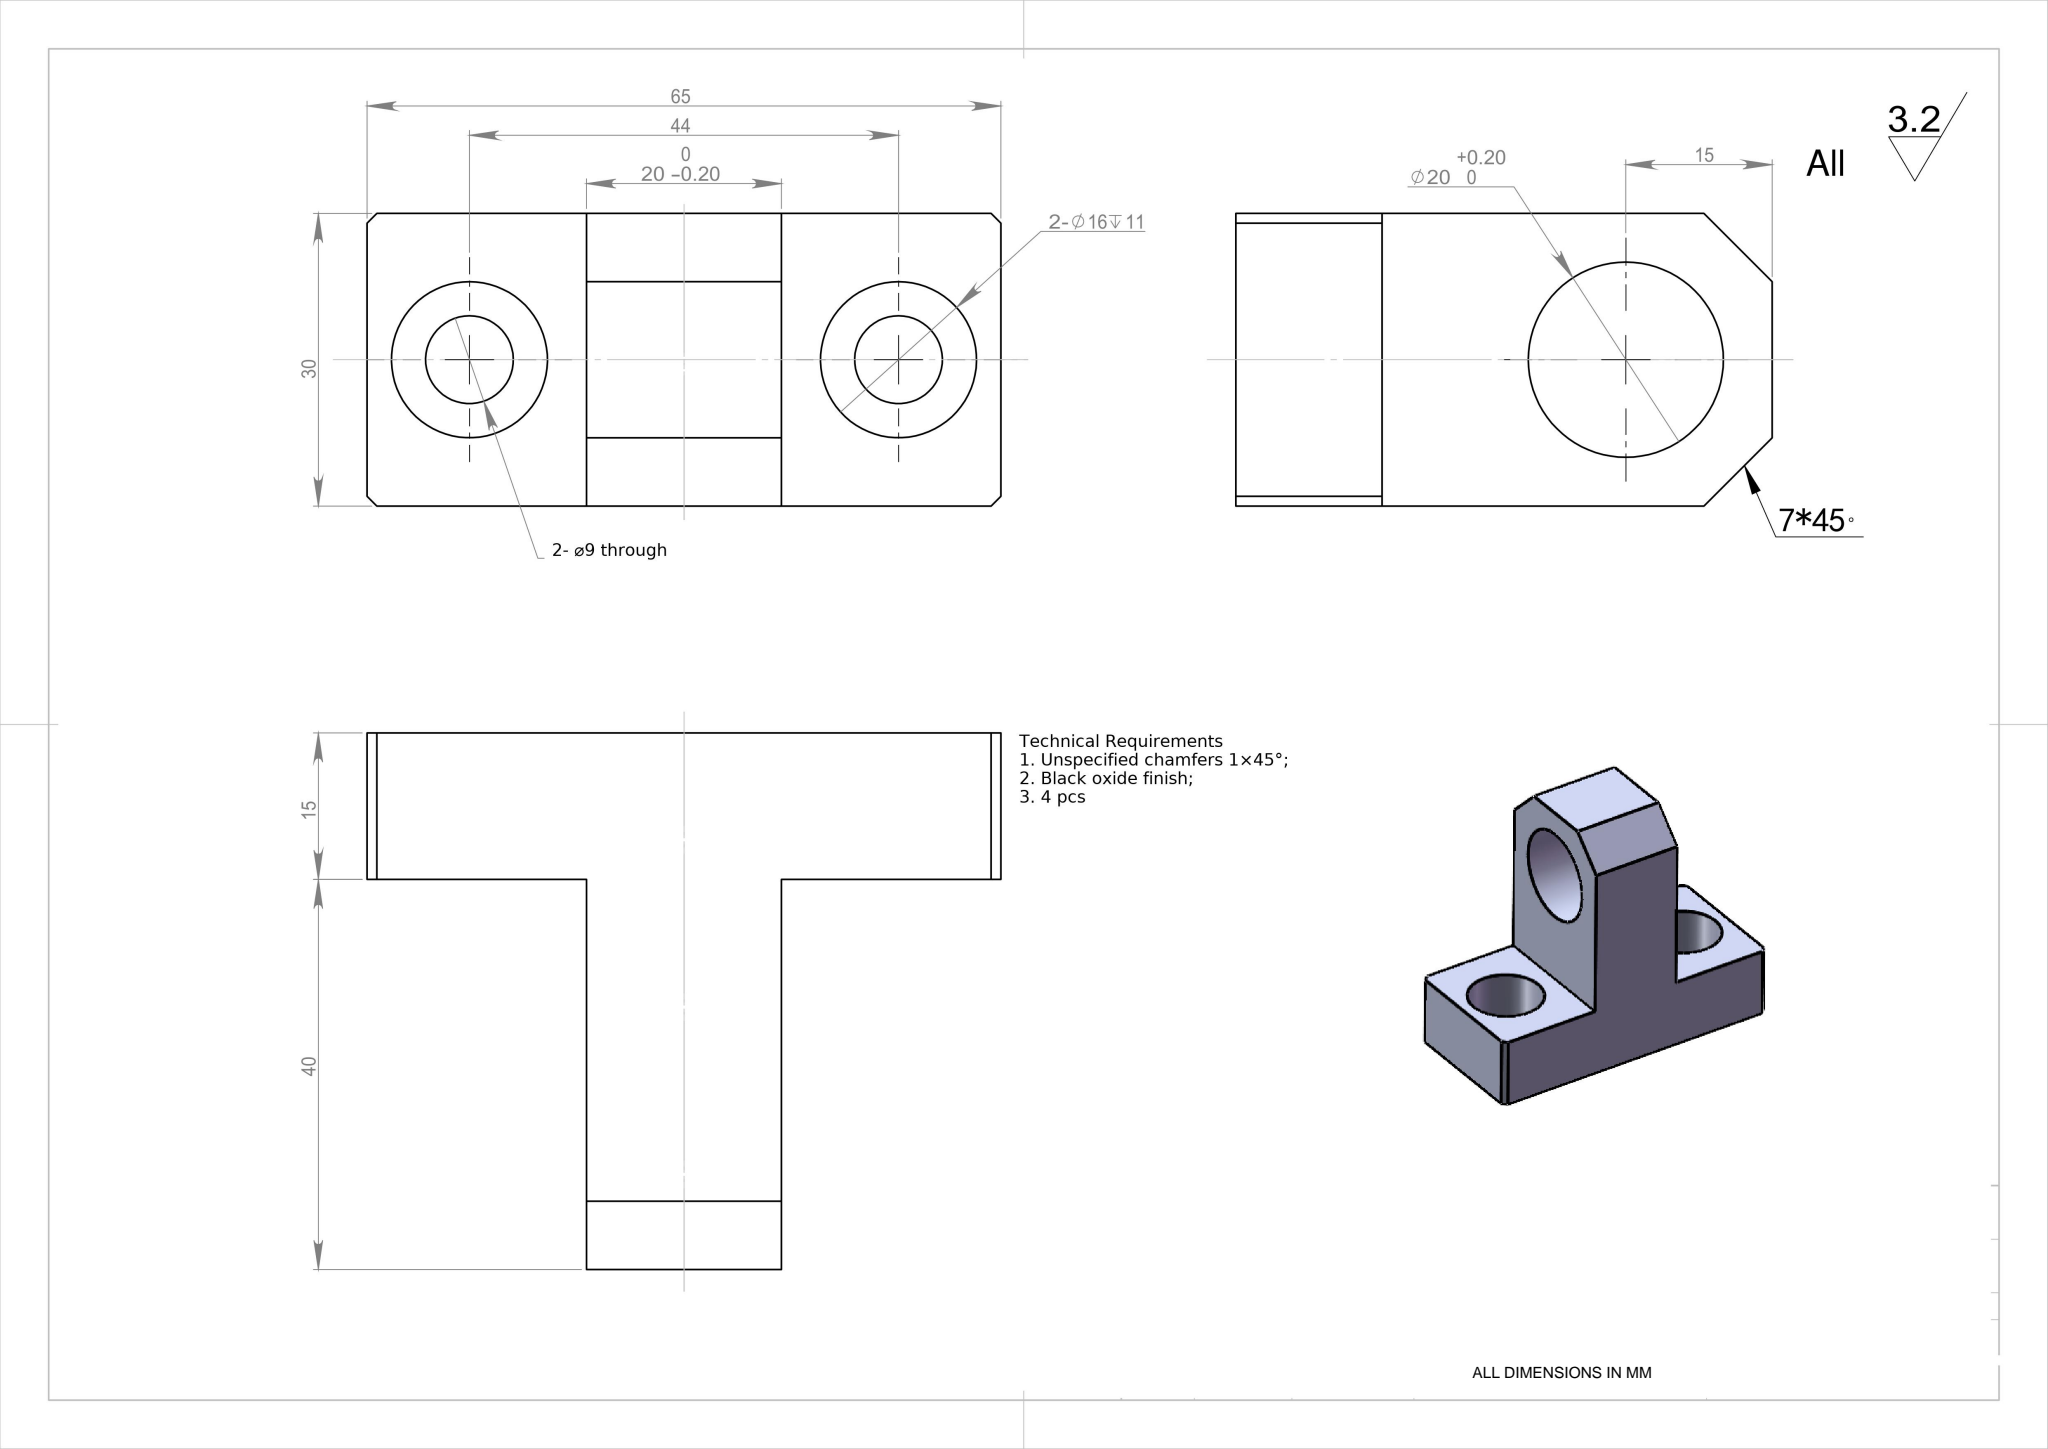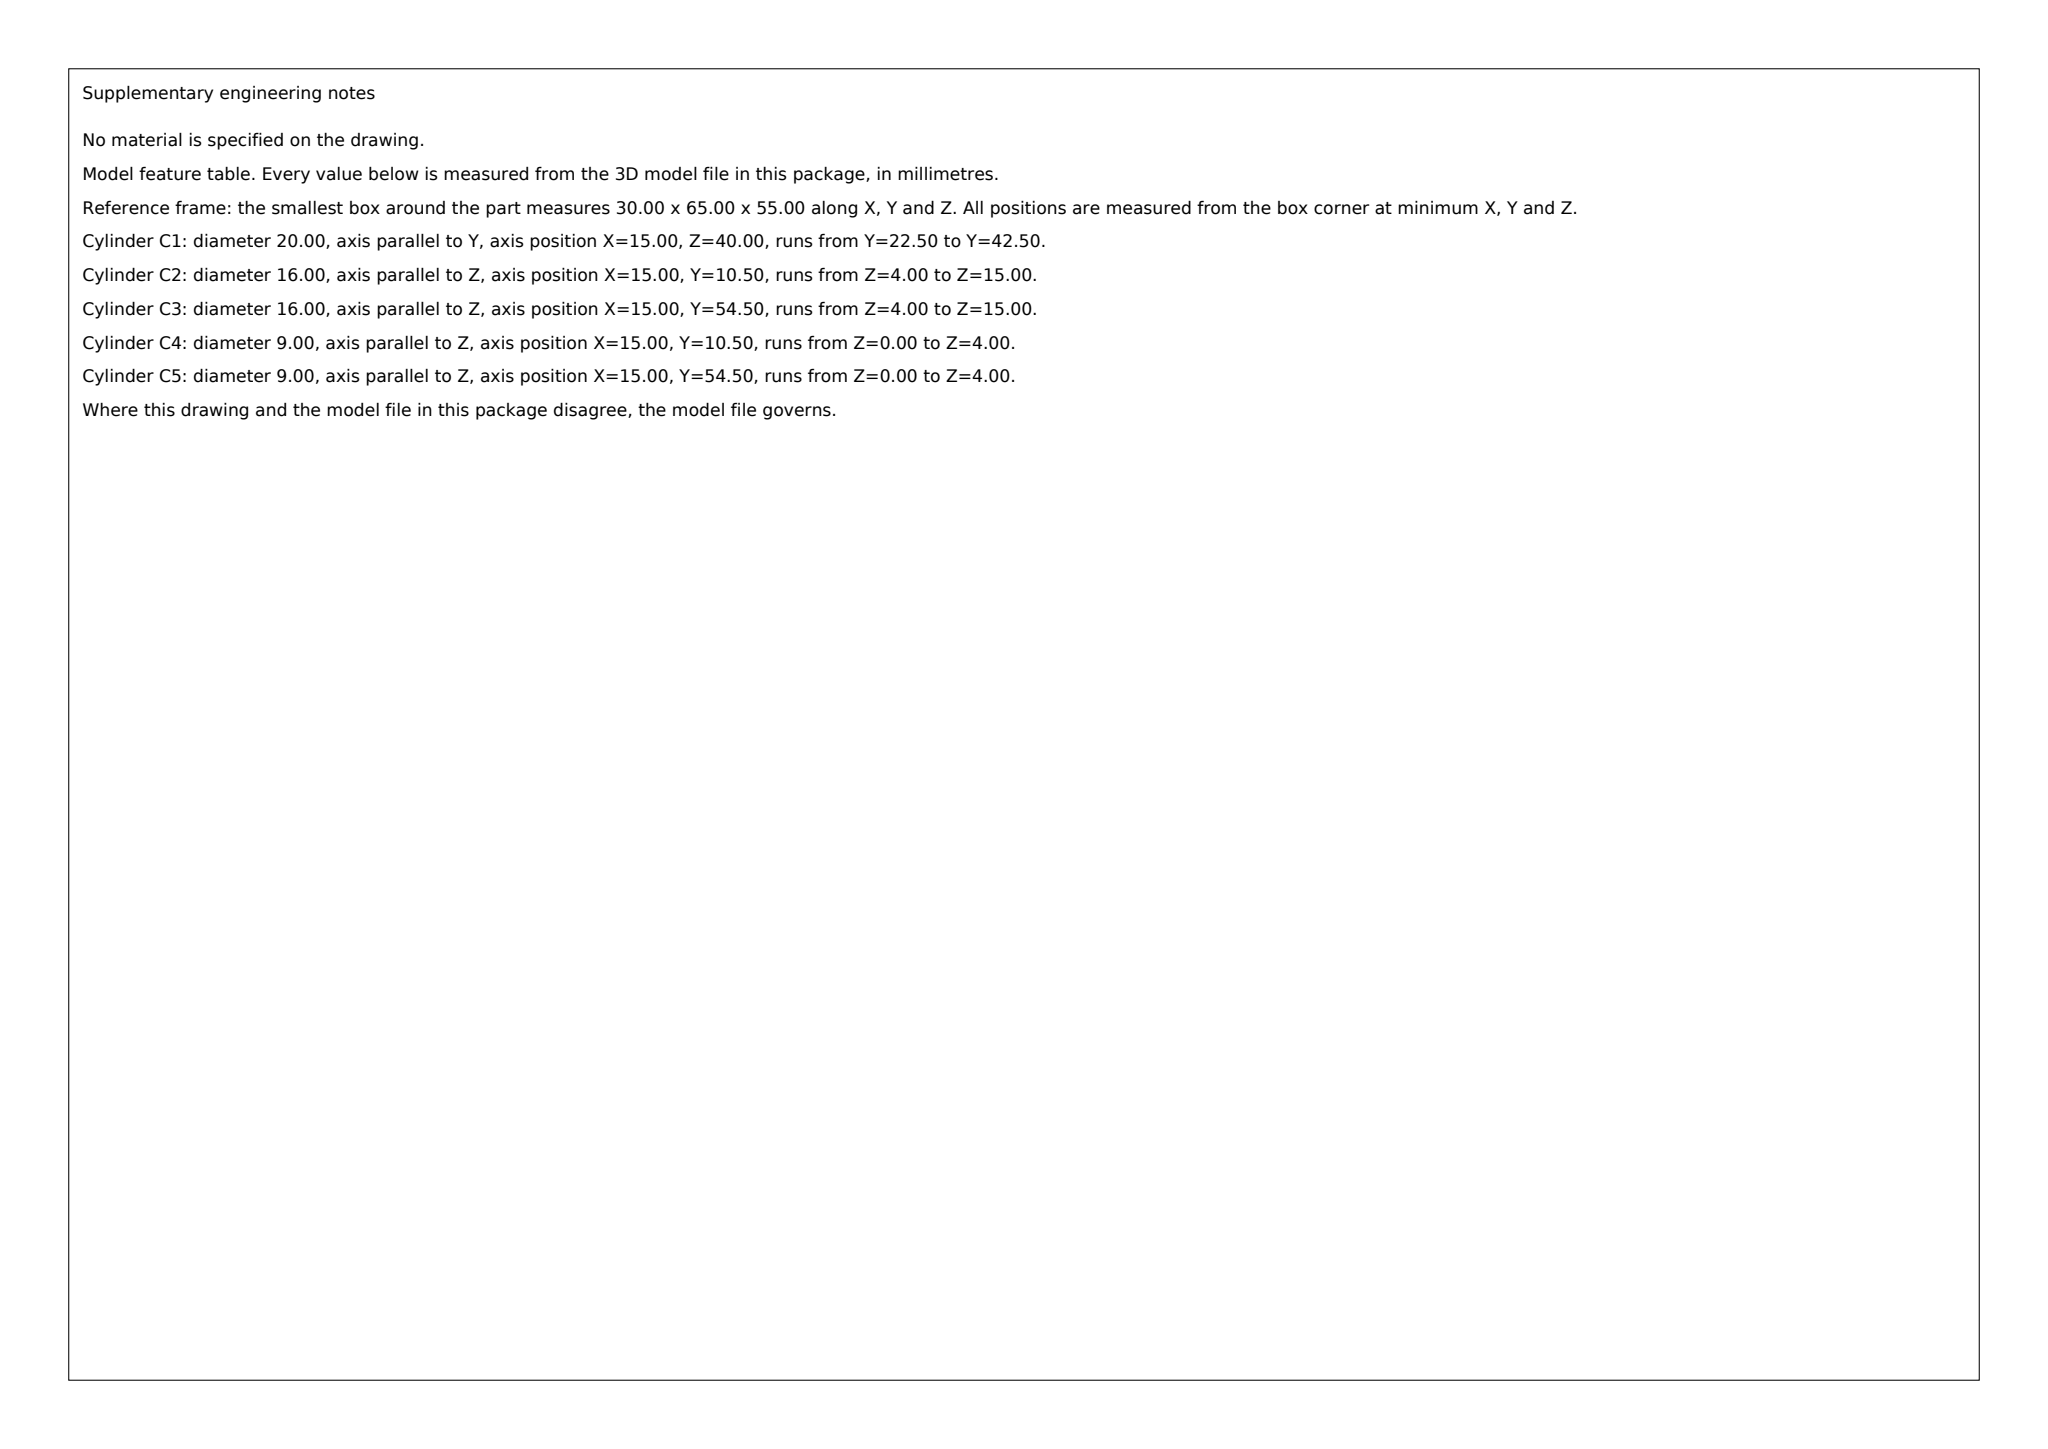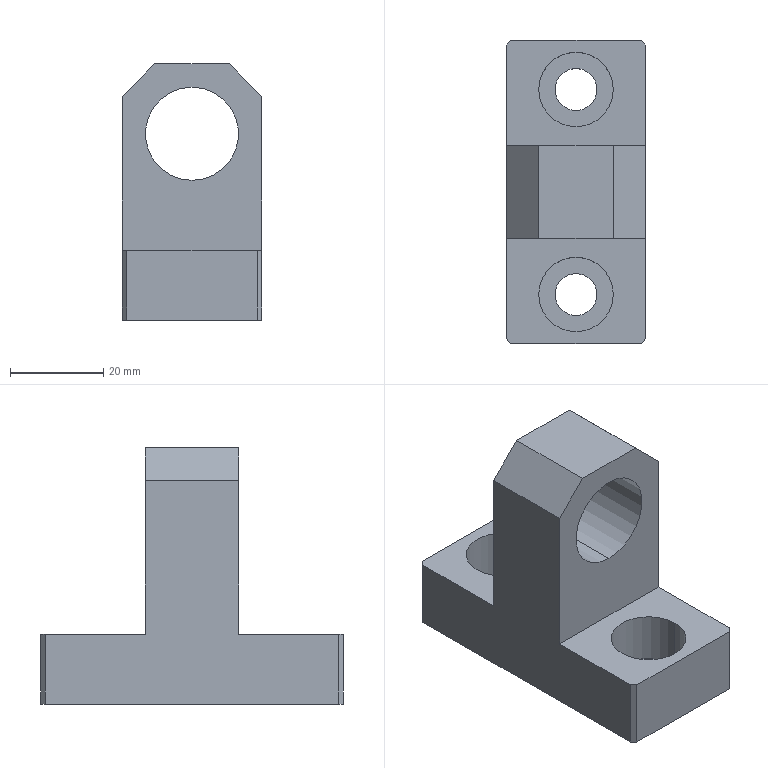Part | SolidWorks | mm | 1 solid | 28 faces | box 30 x 65 x 55 mm | volume 41025 mm3 | plane 18 | cylinder 10 | commonest cylinder face diameters 16 x4 9 x4 20 x2
build123d program:
from build123d import *

# Parameters (mm, degrees)
SKETCH1_W                                         = 30
SKETCH1_H                                         = 20
BOSS_EXTRUDE1_DEPTH                               = 40
SKETCH3_R                                         = 10
CUT_EXTRUDE1_DEPTH                                = 48.17
CHAMFER1_SIZE                                     = 7
SKETCH4_W                                         = 30
SKETCH4_H                                         = 65
BOSS_EXTRUDE3_DEPTH                               = 15
HOLE_SIZE_ACCORDING_TO_HEXAGON_SOCKET_D           = 9
HOLE_SIZE_ACCORDING_TO_HEXAGON_SOCKET_DEPTH       = 35
HOLE_SIZE_ACCORDING_TO_HEXAGON_SOCKET_CBORE_D     = 16
HOLE_SIZE_ACCORDING_TO_HEXAGON_SOCKET_CBORE_DEPTH = 11
HOLE_SIZE_ACCORDING_TO_HEXAGON_SOCKET_TIP         = 2.704
CHAMFER2_SIZE                                     = 1


with BuildPart() as part:
    # Sketch1 → Boss-Extrude1 (new body)
    with BuildSketch(Plane.XY):
        Rectangle(SKETCH1_W, SKETCH1_H)
    extrude(amount=BOSS_EXTRUDE1_DEPTH)

    # Sketch3 → Cut-Extrude1 (cut, through all)
    with BuildSketch(Plane(origin=(0, 10, 0), x_dir=(1, 0, 0), z_dir=(0, 1, 0))):
        with Locations(Location((0, -25, 0), (0, 0, 270))):
            Circle(SKETCH3_R)
    extrude(amount=-CUT_EXTRUDE1_DEPTH, mode=Mode.SUBTRACT)

    # Chamfer1
    chamfer1_edges = [part.edges().sort_by_distance(p)[0] for p in [
        (-15, 0, 40),
        (15, 0, 40),
    ]]
    chamfer(chamfer1_edges, length=CHAMFER1_SIZE)

    # Sketch4 → Boss-Extrude3 (add)
    with BuildSketch(Plane(origin=(0, 0, 0), x_dir=(-1, 0, 0), z_dir=(0, 0, -1))):
        Rectangle(SKETCH4_W, SKETCH4_H)
    extrude(amount=BOSS_EXTRUDE3_DEPTH)

    # Hole Size _ according to_ Hexagon Socket
    with Locations(Plane.XY):
        with Locations((0, 22), (0, -22)):
            CounterBoreHole(HOLE_SIZE_ACCORDING_TO_HEXAGON_SOCKET_D / 2, HOLE_SIZE_ACCORDING_TO_HEXAGON_SOCKET_CBORE_D / 2, HOLE_SIZE_ACCORDING_TO_HEXAGON_SOCKET_CBORE_DEPTH, depth=HOLE_SIZE_ACCORDING_TO_HEXAGON_SOCKET_DEPTH)
            with Locations((0, 0, -(HOLE_SIZE_ACCORDING_TO_HEXAGON_SOCKET_DEPTH + HOLE_SIZE_ACCORDING_TO_HEXAGON_SOCKET_TIP / 2))):  # 118° drill point
                Cone(0, HOLE_SIZE_ACCORDING_TO_HEXAGON_SOCKET_D / 2, HOLE_SIZE_ACCORDING_TO_HEXAGON_SOCKET_TIP, mode=Mode.SUBTRACT)

    # Chamfer2
    chamfer2_edges = [part.edges().sort_by_distance(p)[0] for p in [
        (-15, -32.5, -7.5),
        (-15, 32.5, -7.5),
        (15, 32.5, -7.5),
        (15, -32.5, -7.5),
    ]]
    chamfer(chamfer2_edges, length=CHAMFER2_SIZE)


solid = part.part
STEP:
#1=CARTESIAN_POINT('',(-8.,22.,-11.));
#2=VERTEX_POINT('',#1);
#3=CARTESIAN_POINT('',(8.,22.,-11.));
#4=VERTEX_POINT('',#3);
#5=CARTESIAN_POINT('',(0.,22.,-11.));
#6=DIRECTION('',(0.,0.,1.));
#7=DIRECTION('',(1.,0.,0.));
#8=AXIS2_PLACEMENT_3D('',#5,#6,#7);
#9=CIRCLE('',#8,8.);
#10=EDGE_CURVE('',#2,#4,#9,.T.);
#11=ORIENTED_EDGE('',*,*,#10,.F.);
#12=CARTESIAN_POINT('',(-8.,22.,0.));
#13=VERTEX_POINT('',#12);
#14=CARTESIAN_POINT('',(-8.,22.,0.));
#15=DIRECTION('',(0.,0.,1.));
#16=VECTOR('',#15,1000.);
#17=LINE('',#14,#16);
#18=EDGE_CURVE('',#2,#13,#17,.T.);
#19=ORIENTED_EDGE('',*,*,#18,.T.);
#20=CARTESIAN_POINT('',(8.,22.,0.));
#21=VERTEX_POINT('',#20);
#22=CARTESIAN_POINT('',(0.,22.,0.));
#23=DIRECTION('',(0.,0.,1.));
#24=DIRECTION('',(1.,0.,0.));
#25=AXIS2_PLACEMENT_3D('',#22,#23,#24);
#26=CIRCLE('',#25,8.);
#27=EDGE_CURVE('',#13,#21,#26,.T.);
#28=ORIENTED_EDGE('',*,*,#27,.T.);
#29=CARTESIAN_POINT('',(8.,22.,0.));
#30=DIRECTION('',(0.,0.,1.));
#31=VECTOR('',#30,1000.);
#32=LINE('',#29,#31);
#33=EDGE_CURVE('',#4,#21,#32,.T.);
#34=ORIENTED_EDGE('',*,*,#33,.F.);
#35=EDGE_LOOP('',(#11,#19,#28,#34));
#36=FACE_OUTER_BOUND('',#35,.T.);
#37=CARTESIAN_POINT('',(0.,22.,0.));
#38=DIRECTION('',(0.,0.,1.));
#39=DIRECTION('',(1.,0.,0.));
#40=AXIS2_PLACEMENT_3D('',#37,#38,#39);
#41=CYLINDRICAL_SURFACE('',#40,8.);
#42=ADVANCED_FACE('',(#36),#41,.F.);
#43=CARTESIAN_POINT('',(-4.5,22.,-15.));
#44=VERTEX_POINT('',#43);
#45=CARTESIAN_POINT('',(4.5,22.,-15.));
#46=VERTEX_POINT('',#45);
#47=CARTESIAN_POINT('',(0.,22.,-15.));
#48=DIRECTION('',(0.,0.,1.));
#49=DIRECTION('',(1.,0.,0.));
#50=AXIS2_PLACEMENT_3D('',#47,#48,#49);
#51=CIRCLE('',#50,4.5);
#52=EDGE_CURVE('',#44,#46,#51,.T.);
#53=ORIENTED_EDGE('',*,*,#52,.F.);
#54=CARTESIAN_POINT('',(-4.5,22.,-11.));
#55=VERTEX_POINT('',#54);
#56=CARTESIAN_POINT('',(-4.5,22.,0.));
#57=DIRECTION('',(0.,0.,1.));
#58=VECTOR('',#57,1000.);
#59=LINE('',#56,#58);
#60=EDGE_CURVE('',#44,#55,#59,.T.);
#61=ORIENTED_EDGE('',*,*,#60,.T.);
#62=CARTESIAN_POINT('',(4.5,22.,-11.));
#63=VERTEX_POINT('',#62);
#64=CARTESIAN_POINT('',(0.,22.,-11.));
#65=DIRECTION('',(0.,0.,1.));
#66=DIRECTION('',(1.,0.,0.));
#67=AXIS2_PLACEMENT_3D('',#64,#65,#66);
#68=CIRCLE('',#67,4.5);
#69=EDGE_CURVE('',#55,#63,#68,.T.);
#70=ORIENTED_EDGE('',*,*,#69,.T.);
#71=CARTESIAN_POINT('',(4.5,22.,0.));
#72=DIRECTION('',(0.,0.,1.));
#73=VECTOR('',#72,1000.);
#74=LINE('',#71,#73);
#75=EDGE_CURVE('',#46,#63,#74,.T.);
#76=ORIENTED_EDGE('',*,*,#75,.F.);
#77=EDGE_LOOP('',(#53,#61,#70,#76));
#78=FACE_OUTER_BOUND('',#77,.T.);
#79=CARTESIAN_POINT('',(0.,22.,0.));
#80=DIRECTION('',(0.,0.,1.));
#81=DIRECTION('',(1.,0.,0.));
#82=AXIS2_PLACEMENT_3D('',#79,#80,#81);
#83=CYLINDRICAL_SURFACE('',#82,4.5);
#84=ADVANCED_FACE('',(#78),#83,.F.);
#85=CARTESIAN_POINT('',(-8.,-22.,-11.));
#86=VERTEX_POINT('',#85);
#87=CARTESIAN_POINT('',(8.,-22.,-11.));
#88=VERTEX_POINT('',#87);
#89=CARTESIAN_POINT('',(0.,-22.,-11.));
#90=DIRECTION('',(0.,0.,1.));
#91=DIRECTION('',(1.,0.,0.));
#92=AXIS2_PLACEMENT_3D('',#89,#90,#91);
#93=CIRCLE('',#92,8.);
#94=EDGE_CURVE('',#86,#88,#93,.T.);
#95=ORIENTED_EDGE('',*,*,#94,.F.);
#96=CARTESIAN_POINT('',(-8.,-22.,0.));
#97=VERTEX_POINT('',#96);
#98=CARTESIAN_POINT('',(-8.,-22.,0.));
#99=DIRECTION('',(0.,0.,1.));
#100=VECTOR('',#99,1000.);
#101=LINE('',#98,#100);
#102=EDGE_CURVE('',#86,#97,#101,.T.);
#103=ORIENTED_EDGE('',*,*,#102,.T.);
#104=CARTESIAN_POINT('',(8.,-22.,0.));
#105=VERTEX_POINT('',#104);
#106=CARTESIAN_POINT('',(0.,-22.,0.));
#107=DIRECTION('',(0.,0.,1.));
#108=DIRECTION('',(1.,0.,0.));
#109=AXIS2_PLACEMENT_3D('',#106,#107,#108);
#110=CIRCLE('',#109,8.);
#111=EDGE_CURVE('',#97,#105,#110,.T.);
#112=ORIENTED_EDGE('',*,*,#111,.T.);
#113=CARTESIAN_POINT('',(8.,-22.,0.));
#114=DIRECTION('',(0.,0.,1.));
#115=VECTOR('',#114,1000.);
#116=LINE('',#113,#115);
#117=EDGE_CURVE('',#88,#105,#116,.T.);
#118=ORIENTED_EDGE('',*,*,#117,.F.);
#119=EDGE_LOOP('',(#95,#103,#112,#118));
#120=FACE_OUTER_BOUND('',#119,.T.);
#121=CARTESIAN_POINT('',(0.,-22.,0.));
#122=DIRECTION('',(0.,0.,1.));
#123=DIRECTION('',(1.,0.,0.));
#124=AXIS2_PLACEMENT_3D('',#121,#122,#123);
#125=CYLINDRICAL_SURFACE('',#124,8.);
#126=ADVANCED_FACE('',(#120),#125,.F.);
#127=CARTESIAN_POINT('',(-4.5,-22.,-15.));
#128=VERTEX_POINT('',#127);
#129=CARTESIAN_POINT('',(4.5,-22.,-15.));
#130=VERTEX_POINT('',#129);
#131=CARTESIAN_POINT('',(0.,-22.,-15.));
#132=DIRECTION('',(0.,0.,1.));
#133=DIRECTION('',(1.,0.,0.));
#134=AXIS2_PLACEMENT_3D('',#131,#132,#133);
#135=CIRCLE('',#134,4.5);
#136=EDGE_CURVE('',#128,#130,#135,.T.);
#137=ORIENTED_EDGE('',*,*,#136,.F.);
#138=CARTESIAN_POINT('',(-4.5,-22.,-11.));
#139=VERTEX_POINT('',#138);
#140=CARTESIAN_POINT('',(-4.5,-22.,0.));
#141=DIRECTION('',(0.,0.,1.));
#142=VECTOR('',#141,1000.);
#143=LINE('',#140,#142);
#144=EDGE_CURVE('',#128,#139,#143,.T.);
#145=ORIENTED_EDGE('',*,*,#144,.T.);
#146=CARTESIAN_POINT('',(4.5,-22.,-11.));
#147=VERTEX_POINT('',#146);
#148=CARTESIAN_POINT('',(0.,-22.,-11.));
#149=DIRECTION('',(0.,0.,1.));
#150=DIRECTION('',(1.,0.,0.));
#151=AXIS2_PLACEMENT_3D('',#148,#149,#150);
#152=CIRCLE('',#151,4.5);
#153=EDGE_CURVE('',#139,#147,#152,.T.);
#154=ORIENTED_EDGE('',*,*,#153,.T.);
#155=CARTESIAN_POINT('',(4.5,-22.,0.));
#156=DIRECTION('',(0.,0.,1.));
#157=VECTOR('',#156,1000.);
#158=LINE('',#155,#157);
#159=EDGE_CURVE('',#130,#147,#158,.T.);
#160=ORIENTED_EDGE('',*,*,#159,.F.);
#161=EDGE_LOOP('',(#137,#145,#154,#160));
#162=FACE_OUTER_BOUND('',#161,.T.);
#163=CARTESIAN_POINT('',(0.,-22.,0.));
#164=DIRECTION('',(0.,0.,1.));
#165=DIRECTION('',(1.,0.,0.));
#166=AXIS2_PLACEMENT_3D('',#163,#164,#165);
#167=CYLINDRICAL_SURFACE('',#166,4.5);
#168=ADVANCED_FACE('',(#162),#167,.F.);
#169=CARTESIAN_POINT('',(0.,-10.,15.));
#170=VERTEX_POINT('',#169);
#171=CARTESIAN_POINT('',(0.,-10.,35.));
#172=VERTEX_POINT('',#171);
#173=CARTESIAN_POINT('',(0.,-10.,25.));
#174=DIRECTION('',(0.,1.,0.));
#175=DIRECTION('',(0.,0.,1.));
#176=AXIS2_PLACEMENT_3D('',#173,#174,#175);
#177=CIRCLE('',#176,10.);
#178=EDGE_CURVE('',#170,#172,#177,.T.);
#179=ORIENTED_EDGE('',*,*,#178,.F.);
#180=CARTESIAN_POINT('',(0.,10.,15.));
#181=VERTEX_POINT('',#180);
#182=CARTESIAN_POINT('',(0.,-10.,15.));
#183=DIRECTION('',(0.,1.,0.));
#184=VECTOR('',#183,1000.);
#185=LINE('',#182,#184);
#186=EDGE_CURVE('',#170,#181,#185,.T.);
#187=ORIENTED_EDGE('',*,*,#186,.T.);
#188=CARTESIAN_POINT('',(0.,10.,35.));
#189=VERTEX_POINT('',#188);
#190=CARTESIAN_POINT('',(0.,10.,25.));
#191=DIRECTION('',(0.,1.,0.));
#192=DIRECTION('',(0.,0.,1.));
#193=AXIS2_PLACEMENT_3D('',#190,#191,#192);
#194=CIRCLE('',#193,10.);
#195=EDGE_CURVE('',#181,#189,#194,.T.);
#196=ORIENTED_EDGE('',*,*,#195,.T.);
#197=CARTESIAN_POINT('',(0.,-10.,35.));
#198=DIRECTION('',(0.,1.,0.));
#199=VECTOR('',#198,1000.);
#200=LINE('',#197,#199);
#201=EDGE_CURVE('',#172,#189,#200,.T.);
#202=ORIENTED_EDGE('',*,*,#201,.F.);
#203=EDGE_LOOP('',(#179,#187,#196,#202));
#204=FACE_OUTER_BOUND('',#203,.T.);
#205=CARTESIAN_POINT('',(0.,-10.,25.));
#206=DIRECTION('',(0.,1.,0.));
#207=DIRECTION('',(0.,0.,1.));
#208=AXIS2_PLACEMENT_3D('',#205,#206,#207);
#209=CYLINDRICAL_SURFACE('',#208,10.);
#210=ADVANCED_FACE('',(#204),#209,.F.);
#211=CARTESIAN_POINT('',(15.,-10.,0.));
#212=VERTEX_POINT('',#211);
#213=CARTESIAN_POINT('',(15.,-31.5,0.));
#214=VERTEX_POINT('',#213);
#215=CARTESIAN_POINT('',(15.,-32.5,0.));
#216=DIRECTION('',(0.,-1.,0.));
#217=VECTOR('',#216,1000.);
#218=LINE('',#215,#217);
#219=EDGE_CURVE('',#212,#214,#218,.T.);
#220=ORIENTED_EDGE('',*,*,#219,.T.);
#221=CARTESIAN_POINT('',(15.,-31.5,-15.));
#222=VERTEX_POINT('',#221);
#223=CARTESIAN_POINT('',(15.,-31.5,40.));
#224=DIRECTION('',(0.,0.,-1.));
#225=VECTOR('',#224,1000.);
#226=LINE('',#223,#225);
#227=EDGE_CURVE('',#214,#222,#226,.T.);
#228=ORIENTED_EDGE('',*,*,#227,.T.);
#229=CARTESIAN_POINT('',(15.,31.5,-15.));
#230=VERTEX_POINT('',#229);
#231=CARTESIAN_POINT('',(15.,-32.5,-15.));
#232=DIRECTION('',(0.,-1.,0.));
#233=VECTOR('',#232,1000.);
#234=LINE('',#231,#233);
#235=EDGE_CURVE('',#230,#222,#234,.T.);
#236=ORIENTED_EDGE('',*,*,#235,.F.);
#237=CARTESIAN_POINT('',(15.,31.5,0.));
#238=VERTEX_POINT('',#237);
#239=CARTESIAN_POINT('',(15.,31.5,40.));
#240=DIRECTION('',(0.,0.,1.));
#241=VECTOR('',#240,1000.);
#242=LINE('',#239,#241);
#243=EDGE_CURVE('',#230,#238,#242,.T.);
#244=ORIENTED_EDGE('',*,*,#243,.T.);
#245=CARTESIAN_POINT('',(15.,10.,0.));
#246=VERTEX_POINT('',#245);
#247=CARTESIAN_POINT('',(15.,-32.5,0.));
#248=DIRECTION('',(0.,-1.,0.));
#249=VECTOR('',#248,1000.);
#250=LINE('',#247,#249);
#251=EDGE_CURVE('',#238,#246,#250,.T.);
#252=ORIENTED_EDGE('',*,*,#251,.T.);
#253=CARTESIAN_POINT('',(15.,10.,33.));
#254=VERTEX_POINT('',#253);
#255=CARTESIAN_POINT('',(15.,10.,40.));
#256=DIRECTION('',(0.,0.,-1.));
#257=VECTOR('',#256,1000.);
#258=LINE('',#255,#257);
#259=EDGE_CURVE('',#254,#246,#258,.T.);
#260=ORIENTED_EDGE('',*,*,#259,.F.);
#261=CARTESIAN_POINT('',(15.,-10.,33.));
#262=VERTEX_POINT('',#261);
#263=CARTESIAN_POINT('',(15.,-10.,33.));
#264=DIRECTION('',(0.,-1.,0.));
#265=VECTOR('',#264,1000.);
#266=LINE('',#263,#265);
#267=EDGE_CURVE('',#254,#262,#266,.T.);
#268=ORIENTED_EDGE('',*,*,#267,.T.);
#269=CARTESIAN_POINT('',(15.,-10.,40.));
#270=DIRECTION('',(0.,0.,-1.));
#271=VECTOR('',#270,1000.);
#272=LINE('',#269,#271);
#273=EDGE_CURVE('',#262,#212,#272,.T.);
#274=ORIENTED_EDGE('',*,*,#273,.T.);
#275=EDGE_LOOP('',(#220,#228,#236,#244,#252,#260,#268,#274));
#276=FACE_OUTER_BOUND('',#275,.T.);
#277=CARTESIAN_POINT('',(15.,10.,40.));
#278=DIRECTION('',(-1.,-0.,0.));
#279=DIRECTION('',(0.,-1.,0.));
#280=AXIS2_PLACEMENT_3D('',#277,#278,#279);
#281=PLANE('',#280);
#282=ADVANCED_FACE('',(#276),#281,.F.);
#283=CARTESIAN_POINT('',(0.,10.,25.));
#284=DIRECTION('',(0.,1.,0.));
#285=DIRECTION('',(0.,0.,1.));
#286=AXIS2_PLACEMENT_3D('',#283,#284,#285);
#287=CIRCLE('',#286,10.);
#288=EDGE_CURVE('',#189,#181,#287,.T.);
#289=ORIENTED_EDGE('',*,*,#288,.F.);
#290=ORIENTED_EDGE('',*,*,#195,.F.);
#291=EDGE_LOOP('',(#289,#290));
#292=FACE_BOUND('',#291,.T.);
#293=CARTESIAN_POINT('',(8.,10.,40.));
#294=VERTEX_POINT('',#293);
#295=CARTESIAN_POINT('',(-8.,10.,40.));
#296=VERTEX_POINT('',#295);
#297=CARTESIAN_POINT('',(-15.,10.,40.));
#298=DIRECTION('',(-1.,0.,0.));
#299=VECTOR('',#298,1000.);
#300=LINE('',#297,#299);
#301=EDGE_CURVE('',#294,#296,#300,.T.);
#302=ORIENTED_EDGE('',*,*,#301,.F.);
#303=CARTESIAN_POINT('',(8.,10.,40.));
#304=DIRECTION('',(0.7071,0.,-0.7071));
#305=VECTOR('',#304,1000.);
#306=LINE('',#303,#305);
#307=EDGE_CURVE('',#294,#254,#306,.T.);
#308=ORIENTED_EDGE('',*,*,#307,.T.);
#309=ORIENTED_EDGE('',*,*,#259,.T.);
#310=CARTESIAN_POINT('',(-15.,10.,0.));
#311=VERTEX_POINT('',#310);
#312=CARTESIAN_POINT('',(-15.,10.,0.));
#313=DIRECTION('',(-1.,0.,0.));
#314=VECTOR('',#313,1000.);
#315=LINE('',#312,#314);
#316=EDGE_CURVE('',#246,#311,#315,.T.);
#317=ORIENTED_EDGE('',*,*,#316,.T.);
#318=CARTESIAN_POINT('',(-15.,10.,33.));
#319=VERTEX_POINT('',#318);
#320=CARTESIAN_POINT('',(-15.,10.,40.));
#321=DIRECTION('',(0.,0.,-1.));
#322=VECTOR('',#321,1000.);
#323=LINE('',#320,#322);
#324=EDGE_CURVE('',#319,#311,#323,.T.);
#325=ORIENTED_EDGE('',*,*,#324,.F.);
#326=CARTESIAN_POINT('',(-8.,10.,40.));
#327=DIRECTION('',(0.7071,0.,0.7071));
#328=VECTOR('',#327,1000.);
#329=LINE('',#326,#328);
#330=EDGE_CURVE('',#319,#296,#329,.T.);
#331=ORIENTED_EDGE('',*,*,#330,.T.);
#332=EDGE_LOOP('',(#302,#308,#309,#317,#325,#331));
#333=FACE_OUTER_BOUND('',#332,.T.);
#334=CARTESIAN_POINT('',(-15.,10.,40.));
#335=DIRECTION('',(0.,-1.,0.));
#336=DIRECTION('',(0.,0.,-1.));
#337=AXIS2_PLACEMENT_3D('',#334,#335,#336);
#338=PLANE('',#337);
#339=ADVANCED_FACE('',(#292,#333),#338,.F.);
#340=CARTESIAN_POINT('',(-15.,-31.5,-15.));
#341=VERTEX_POINT('',#340);
#342=CARTESIAN_POINT('',(-15.,31.5,-15.));
#343=VERTEX_POINT('',#342);
#344=CARTESIAN_POINT('',(-15.,-32.5,-15.));
#345=DIRECTION('',(0.,1.,0.));
#346=VECTOR('',#345,1000.);
#347=LINE('',#344,#346);
#348=EDGE_CURVE('',#341,#343,#347,.T.);
#349=ORIENTED_EDGE('',*,*,#348,.F.);
#350=CARTESIAN_POINT('',(-15.,-31.5,0.));
#351=VERTEX_POINT('',#350);
#352=CARTESIAN_POINT('',(-15.,-31.5,40.));
#353=DIRECTION('',(0.,0.,1.));
#354=VECTOR('',#353,1000.);
#355=LINE('',#352,#354);
#356=EDGE_CURVE('',#341,#351,#355,.T.);
#357=ORIENTED_EDGE('',*,*,#356,.T.);
#358=CARTESIAN_POINT('',(-15.,-10.,0.));
#359=VERTEX_POINT('',#358);
#360=CARTESIAN_POINT('',(-15.,-32.5,0.));
#361=DIRECTION('',(0.,1.,0.));
#362=VECTOR('',#361,1000.);
#363=LINE('',#360,#362);
#364=EDGE_CURVE('',#351,#359,#363,.T.);
#365=ORIENTED_EDGE('',*,*,#364,.T.);
#366=CARTESIAN_POINT('',(-15.,-10.,33.));
#367=VERTEX_POINT('',#366);
#368=CARTESIAN_POINT('',(-15.,-10.,40.));
#369=DIRECTION('',(0.,0.,-1.));
#370=VECTOR('',#369,1000.);
#371=LINE('',#368,#370);
#372=EDGE_CURVE('',#367,#359,#371,.T.);
#373=ORIENTED_EDGE('',*,*,#372,.F.);
#374=CARTESIAN_POINT('',(-15.,10.,33.));
#375=DIRECTION('',(-0.,1.,0.));
#376=VECTOR('',#375,1000.);
#377=LINE('',#374,#376);
#378=EDGE_CURVE('',#367,#319,#377,.T.);
#379=ORIENTED_EDGE('',*,*,#378,.T.);
#380=ORIENTED_EDGE('',*,*,#324,.T.);
#381=CARTESIAN_POINT('',(-15.,31.5,0.));
#382=VERTEX_POINT('',#381);
#383=CARTESIAN_POINT('',(-15.,-32.5,0.));
#384=DIRECTION('',(0.,1.,0.));
#385=VECTOR('',#384,1000.);
#386=LINE('',#383,#385);
#387=EDGE_CURVE('',#311,#382,#386,.T.);
#388=ORIENTED_EDGE('',*,*,#387,.T.);
#389=CARTESIAN_POINT('',(-15.,31.5,40.));
#390=DIRECTION('',(0.,0.,-1.));
#391=VECTOR('',#390,1000.);
#392=LINE('',#389,#391);
#393=EDGE_CURVE('',#382,#343,#392,.T.);
#394=ORIENTED_EDGE('',*,*,#393,.T.);
#395=EDGE_LOOP('',(#349,#357,#365,#373,#379,#380,#388,#394));
#396=FACE_OUTER_BOUND('',#395,.T.);
#397=CARTESIAN_POINT('',(-15.,10.,40.));
#398=DIRECTION('',(1.,0.,0.));
#399=DIRECTION('',(-0.,1.,0.));
#400=AXIS2_PLACEMENT_3D('',#397,#398,#399);
#401=PLANE('',#400);
#402=ADVANCED_FACE('',(#396),#401,.F.);
#403=CARTESIAN_POINT('',(0.,-10.,25.));
#404=DIRECTION('',(0.,1.,0.));
#405=DIRECTION('',(0.,0.,1.));
#406=AXIS2_PLACEMENT_3D('',#403,#404,#405);
#407=CIRCLE('',#406,10.);
#408=EDGE_CURVE('',#172,#170,#407,.T.);
#409=ORIENTED_EDGE('',*,*,#408,.T.);
#410=ORIENTED_EDGE('',*,*,#178,.T.);
#411=EDGE_LOOP('',(#409,#410));
#412=FACE_BOUND('',#411,.T.);
#413=ORIENTED_EDGE('',*,*,#273,.F.);
#414=CARTESIAN_POINT('',(8.,-10.,40.));
#415=VERTEX_POINT('',#414);
#416=CARTESIAN_POINT('',(8.,-10.,40.));
#417=DIRECTION('',(-0.7071,0.,0.7071));
#418=VECTOR('',#417,1000.);
#419=LINE('',#416,#418);
#420=EDGE_CURVE('',#262,#415,#419,.T.);
#421=ORIENTED_EDGE('',*,*,#420,.T.);
#422=CARTESIAN_POINT('',(-8.,-10.,40.));
#423=VERTEX_POINT('',#422);
#424=CARTESIAN_POINT('',(-15.,-10.,40.));
#425=DIRECTION('',(1.,0.,0.));
#426=VECTOR('',#425,1000.);
#427=LINE('',#424,#426);
#428=EDGE_CURVE('',#423,#415,#427,.T.);
#429=ORIENTED_EDGE('',*,*,#428,.F.);
#430=CARTESIAN_POINT('',(-8.,-10.,40.));
#431=DIRECTION('',(-0.7071,0.,-0.7071));
#432=VECTOR('',#431,1000.);
#433=LINE('',#430,#432);
#434=EDGE_CURVE('',#423,#367,#433,.T.);
#435=ORIENTED_EDGE('',*,*,#434,.T.);
#436=ORIENTED_EDGE('',*,*,#372,.T.);
#437=CARTESIAN_POINT('',(-15.,-10.,0.));
#438=DIRECTION('',(1.,0.,0.));
#439=VECTOR('',#438,1000.);
#440=LINE('',#437,#439);
#441=EDGE_CURVE('',#359,#212,#440,.T.);
#442=ORIENTED_EDGE('',*,*,#441,.T.);
#443=EDGE_LOOP('',(#413,#421,#429,#435,#436,#442));
#444=FACE_OUTER_BOUND('',#443,.T.);
#445=CARTESIAN_POINT('',(-15.,-10.,40.));
#446=DIRECTION('',(0.,1.,0.));
#447=DIRECTION('',(0.,0.,1.));
#448=AXIS2_PLACEMENT_3D('',#445,#446,#447);
#449=PLANE('',#448);
#450=ADVANCED_FACE('',(#412,#444),#449,.F.);
#451=ORIENTED_EDGE('',*,*,#428,.T.);
#452=CARTESIAN_POINT('',(8.,10.,40.));
#453=DIRECTION('',(-0.,1.,0.));
#454=VECTOR('',#453,1000.);
#455=LINE('',#452,#454);
#456=EDGE_CURVE('',#415,#294,#455,.T.);
#457=ORIENTED_EDGE('',*,*,#456,.T.);
#458=ORIENTED_EDGE('',*,*,#301,.T.);
#459=CARTESIAN_POINT('',(-8.,-10.,40.));
#460=DIRECTION('',(0.,-1.,0.));
#461=VECTOR('',#460,1000.);
#462=LINE('',#459,#461);
#463=EDGE_CURVE('',#296,#423,#462,.T.);
#464=ORIENTED_EDGE('',*,*,#463,.T.);
#465=EDGE_LOOP('',(#451,#457,#458,#464));
#466=FACE_OUTER_BOUND('',#465,.T.);
#467=CARTESIAN_POINT('',(0.,0.,40.));
#468=DIRECTION('',(0.,0.,1.));
#469=DIRECTION('',(1.,0.,0.));
#470=AXIS2_PLACEMENT_3D('',#467,#468,#469);
#471=PLANE('',#470);
#472=ADVANCED_FACE('',(#466),#471,.T.);
#473=ORIENTED_EDGE('',*,*,#186,.F.);
#474=ORIENTED_EDGE('',*,*,#408,.F.);
#475=ORIENTED_EDGE('',*,*,#201,.T.);
#476=ORIENTED_EDGE('',*,*,#288,.T.);
#477=EDGE_LOOP('',(#473,#474,#475,#476));
#478=FACE_OUTER_BOUND('',#477,.T.);
#479=CARTESIAN_POINT('',(0.,-10.,25.));
#480=DIRECTION('',(0.,1.,0.));
#481=DIRECTION('',(0.,0.,1.));
#482=AXIS2_PLACEMENT_3D('',#479,#480,#481);
#483=CYLINDRICAL_SURFACE('',#482,10.);
#484=ADVANCED_FACE('',(#478),#483,.F.);
#485=ORIENTED_EDGE('',*,*,#420,.F.);
#486=ORIENTED_EDGE('',*,*,#267,.F.);
#487=ORIENTED_EDGE('',*,*,#307,.F.);
#488=ORIENTED_EDGE('',*,*,#456,.F.);
#489=EDGE_LOOP('',(#485,#486,#487,#488));
#490=FACE_OUTER_BOUND('',#489,.T.);
#491=CARTESIAN_POINT('',(8.,0.,40.));
#492=DIRECTION('',(0.7071,0.,0.7071));
#493=DIRECTION('',(0.,-1.,0.));
#494=AXIS2_PLACEMENT_3D('',#491,#492,#493);
#495=PLANE('',#494);
#496=ADVANCED_FACE('',(#490),#495,.T.);
#497=ORIENTED_EDGE('',*,*,#330,.F.);
#498=ORIENTED_EDGE('',*,*,#378,.F.);
#499=ORIENTED_EDGE('',*,*,#434,.F.);
#500=ORIENTED_EDGE('',*,*,#463,.F.);
#501=EDGE_LOOP('',(#497,#498,#499,#500));
#502=FACE_OUTER_BOUND('',#501,.T.);
#503=CARTESIAN_POINT('',(-8.,-0.,40.));
#504=DIRECTION('',(-0.7071,-0.,0.7071));
#505=DIRECTION('',(-0.,1.,0.));
#506=AXIS2_PLACEMENT_3D('',#503,#504,#505);
#507=PLANE('',#506);
#508=ADVANCED_FACE('',(#502),#507,.T.);
#509=CARTESIAN_POINT('',(0.,-22.,0.));
#510=DIRECTION('',(0.,0.,1.));
#511=DIRECTION('',(1.,0.,0.));
#512=AXIS2_PLACEMENT_3D('',#509,#510,#511);
#513=CIRCLE('',#512,8.);
#514=EDGE_CURVE('',#105,#97,#513,.T.);
#515=ORIENTED_EDGE('',*,*,#514,.F.);
#516=ORIENTED_EDGE('',*,*,#111,.F.);
#517=EDGE_LOOP('',(#515,#516));
#518=FACE_BOUND('',#517,.T.);
#519=CARTESIAN_POINT('',(14.,-32.5,0.));
#520=VERTEX_POINT('',#519);
#521=CARTESIAN_POINT('',(-14.,-32.5,0.));
#522=VERTEX_POINT('',#521);
#523=CARTESIAN_POINT('',(15.,-32.5,0.));
#524=DIRECTION('',(-1.,0.,0.));
#525=VECTOR('',#524,1000.);
#526=LINE('',#523,#525);
#527=EDGE_CURVE('',#520,#522,#526,.T.);
#528=ORIENTED_EDGE('',*,*,#527,.F.);
#529=CARTESIAN_POINT('',(23.25,-23.25,0.));
#530=DIRECTION('',(0.7071,0.7071,0.));
#531=VECTOR('',#530,1000.);
#532=LINE('',#529,#531);
#533=EDGE_CURVE('',#520,#214,#532,.T.);
#534=ORIENTED_EDGE('',*,*,#533,.T.);
#535=ORIENTED_EDGE('',*,*,#219,.F.);
#536=ORIENTED_EDGE('',*,*,#441,.F.);
#537=ORIENTED_EDGE('',*,*,#364,.F.);
#538=CARTESIAN_POINT('',(-23.25,-23.25,0.));
#539=DIRECTION('',(0.7071,-0.7071,0.));
#540=VECTOR('',#539,1000.);
#541=LINE('',#538,#540);
#542=EDGE_CURVE('',#351,#522,#541,.T.);
#543=ORIENTED_EDGE('',*,*,#542,.T.);
#544=EDGE_LOOP('',(#528,#534,#535,#536,#537,#543));
#545=FACE_OUTER_BOUND('',#544,.T.);
#546=CARTESIAN_POINT('',(0.,0.,0.));
#547=DIRECTION('',(0.,0.,1.));
#548=DIRECTION('',(1.,0.,0.));
#549=AXIS2_PLACEMENT_3D('',#546,#547,#548);
#550=PLANE('',#549);
#551=ADVANCED_FACE('',(#518,#545),#550,.T.);
#552=CARTESIAN_POINT('',(0.,22.,0.));
#553=DIRECTION('',(0.,0.,1.));
#554=DIRECTION('',(1.,0.,0.));
#555=AXIS2_PLACEMENT_3D('',#552,#553,#554);
#556=CIRCLE('',#555,8.);
#557=EDGE_CURVE('',#21,#13,#556,.T.);
#558=ORIENTED_EDGE('',*,*,#557,.F.);
#559=ORIENTED_EDGE('',*,*,#27,.F.);
#560=EDGE_LOOP('',(#558,#559));
#561=FACE_BOUND('',#560,.T.);
#562=ORIENTED_EDGE('',*,*,#251,.F.);
#563=CARTESIAN_POINT('',(14.,32.5,0.));
#564=VERTEX_POINT('',#563);
#565=CARTESIAN_POINT('',(23.25,23.25,0.));
#566=DIRECTION('',(-0.7071,0.7071,0.));
#567=VECTOR('',#566,1000.);
#568=LINE('',#565,#567);
#569=EDGE_CURVE('',#238,#564,#568,.T.);
#570=ORIENTED_EDGE('',*,*,#569,.T.);
#571=CARTESIAN_POINT('',(-14.,32.5,0.));
#572=VERTEX_POINT('',#571);
#573=CARTESIAN_POINT('',(15.,32.5,0.));
#574=DIRECTION('',(1.,0.,0.));
#575=VECTOR('',#574,1000.);
#576=LINE('',#573,#575);
#577=EDGE_CURVE('',#572,#564,#576,.T.);
#578=ORIENTED_EDGE('',*,*,#577,.F.);
#579=CARTESIAN_POINT('',(-23.25,23.25,0.));
#580=DIRECTION('',(-0.7071,-0.7071,0.));
#581=VECTOR('',#580,1000.);
#582=LINE('',#579,#581);
#583=EDGE_CURVE('',#572,#382,#582,.T.);
#584=ORIENTED_EDGE('',*,*,#583,.T.);
#585=ORIENTED_EDGE('',*,*,#387,.F.);
#586=ORIENTED_EDGE('',*,*,#316,.F.);
#587=EDGE_LOOP('',(#562,#570,#578,#584,#585,#586));
#588=FACE_OUTER_BOUND('',#587,.T.);
#589=CARTESIAN_POINT('',(0.,0.,0.));
#590=DIRECTION('',(0.,0.,1.));
#591=DIRECTION('',(1.,0.,0.));
#592=AXIS2_PLACEMENT_3D('',#589,#590,#591);
#593=PLANE('',#592);
#594=ADVANCED_FACE('',(#561,#588),#593,.T.);
#595=ORIENTED_EDGE('',*,*,#577,.T.);
#596=CARTESIAN_POINT('',(14.,32.5,-15.));
#597=VERTEX_POINT('',#596);
#598=CARTESIAN_POINT('',(14.,32.5,-15.));
#599=DIRECTION('',(0.,0.,-1.));
#600=VECTOR('',#599,1000.);
#601=LINE('',#598,#600);
#602=EDGE_CURVE('',#564,#597,#601,.T.);
#603=ORIENTED_EDGE('',*,*,#602,.T.);
#604=CARTESIAN_POINT('',(-14.,32.5,-15.));
#605=VERTEX_POINT('',#604);
#606=CARTESIAN_POINT('',(15.,32.5,-15.));
#607=DIRECTION('',(1.,0.,0.));
#608=VECTOR('',#607,1000.);
#609=LINE('',#606,#608);
#610=EDGE_CURVE('',#605,#597,#609,.T.);
#611=ORIENTED_EDGE('',*,*,#610,.F.);
#612=CARTESIAN_POINT('',(-14.,32.5,-15.));
#613=DIRECTION('',(0.,0.,1.));
#614=VECTOR('',#613,1000.);
#615=LINE('',#612,#614);
#616=EDGE_CURVE('',#605,#572,#615,.T.);
#617=ORIENTED_EDGE('',*,*,#616,.T.);
#618=EDGE_LOOP('',(#595,#603,#611,#617));
#619=FACE_OUTER_BOUND('',#618,.T.);
#620=CARTESIAN_POINT('',(15.,32.5,-15.));
#621=DIRECTION('',(0.,-1.,0.));
#622=DIRECTION('',(0.,0.,-1.));
#623=AXIS2_PLACEMENT_3D('',#620,#621,#622);
#624=PLANE('',#623);
#625=ADVANCED_FACE('',(#619),#624,.F.);
#626=CARTESIAN_POINT('',(14.,-32.5,-15.));
#627=VERTEX_POINT('',#626);
#628=CARTESIAN_POINT('',(-14.,-32.5,-15.));
#629=VERTEX_POINT('',#628);
#630=CARTESIAN_POINT('',(15.,-32.5,-15.));
#631=DIRECTION('',(-1.,0.,0.));
#632=VECTOR('',#631,1000.);
#633=LINE('',#630,#632);
#634=EDGE_CURVE('',#627,#629,#633,.T.);
#635=ORIENTED_EDGE('',*,*,#634,.F.);
#636=CARTESIAN_POINT('',(14.,-32.5,-15.));
#637=DIRECTION('',(0.,0.,1.));
#638=VECTOR('',#637,1000.);
#639=LINE('',#636,#638);
#640=EDGE_CURVE('',#627,#520,#639,.T.);
#641=ORIENTED_EDGE('',*,*,#640,.T.);
#642=ORIENTED_EDGE('',*,*,#527,.T.);
#643=CARTESIAN_POINT('',(-14.,-32.5,-15.));
#644=DIRECTION('',(0.,0.,-1.));
#645=VECTOR('',#644,1000.);
#646=LINE('',#643,#645);
#647=EDGE_CURVE('',#522,#629,#646,.T.);
#648=ORIENTED_EDGE('',*,*,#647,.T.);
#649=EDGE_LOOP('',(#635,#641,#642,#648));
#650=FACE_OUTER_BOUND('',#649,.T.);
#651=CARTESIAN_POINT('',(15.,-32.5,-15.));
#652=DIRECTION('',(0.,1.,0.));
#653=DIRECTION('',(0.,0.,1.));
#654=AXIS2_PLACEMENT_3D('',#651,#652,#653);
#655=PLANE('',#654);
#656=ADVANCED_FACE('',(#650),#655,.F.);
#657=CARTESIAN_POINT('',(0.,22.,-15.));
#658=DIRECTION('',(0.,0.,1.));
#659=DIRECTION('',(1.,0.,0.));
#660=AXIS2_PLACEMENT_3D('',#657,#658,#659);
#661=CIRCLE('',#660,4.5);
#662=EDGE_CURVE('',#46,#44,#661,.T.);
#663=ORIENTED_EDGE('',*,*,#662,.T.);
#664=ORIENTED_EDGE('',*,*,#52,.T.);
#665=EDGE_LOOP('',(#663,#664));
#666=FACE_BOUND('',#665,.T.);
#667=CARTESIAN_POINT('',(0.,-22.,-15.));
#668=DIRECTION('',(0.,0.,1.));
#669=DIRECTION('',(1.,0.,0.));
#670=AXIS2_PLACEMENT_3D('',#667,#668,#669);
#671=CIRCLE('',#670,4.5);
#672=EDGE_CURVE('',#130,#128,#671,.T.);
#673=ORIENTED_EDGE('',*,*,#672,.T.);
#674=ORIENTED_EDGE('',*,*,#136,.T.);
#675=EDGE_LOOP('',(#673,#674));
#676=FACE_BOUND('',#675,.T.);
#677=ORIENTED_EDGE('',*,*,#235,.T.);
#678=CARTESIAN_POINT('',(14.,-32.5,-15.));
#679=DIRECTION('',(-0.7071,-0.7071,0.));
#680=VECTOR('',#679,1000.);
#681=LINE('',#678,#680);
#682=EDGE_CURVE('',#222,#627,#681,.T.);
#683=ORIENTED_EDGE('',*,*,#682,.T.);
#684=ORIENTED_EDGE('',*,*,#634,.T.);
#685=CARTESIAN_POINT('',(-15.,-31.5,-15.));
#686=DIRECTION('',(-0.7071,0.7071,0.));
#687=VECTOR('',#686,1000.);
#688=LINE('',#685,#687);
#689=EDGE_CURVE('',#629,#341,#688,.T.);
#690=ORIENTED_EDGE('',*,*,#689,.T.);
#691=ORIENTED_EDGE('',*,*,#348,.T.);
#692=CARTESIAN_POINT('',(-14.,32.5,-15.));
#693=DIRECTION('',(0.7071,0.7071,0.));
#694=VECTOR('',#693,1000.);
#695=LINE('',#692,#694);
#696=EDGE_CURVE('',#343,#605,#695,.T.);
#697=ORIENTED_EDGE('',*,*,#696,.T.);
#698=ORIENTED_EDGE('',*,*,#610,.T.);
#699=CARTESIAN_POINT('',(15.,31.5,-15.));
#700=DIRECTION('',(0.7071,-0.7071,0.));
#701=VECTOR('',#700,1000.);
#702=LINE('',#699,#701);
#703=EDGE_CURVE('',#597,#230,#702,.T.);
#704=ORIENTED_EDGE('',*,*,#703,.T.);
#705=EDGE_LOOP('',(#677,#683,#684,#690,#691,#697,#698,#704));
#706=FACE_OUTER_BOUND('',#705,.T.);
#707=CARTESIAN_POINT('',(0.,0.,-15.));
#708=DIRECTION('',(0.,0.,1.));
#709=DIRECTION('',(1.,0.,0.));
#710=AXIS2_PLACEMENT_3D('',#707,#708,#709);
#711=PLANE('',#710);
#712=ADVANCED_FACE('',(#666,#676,#706),#711,.F.);
#713=ORIENTED_EDGE('',*,*,#144,.F.);
#714=ORIENTED_EDGE('',*,*,#672,.F.);
#715=ORIENTED_EDGE('',*,*,#159,.T.);
#716=CARTESIAN_POINT('',(0.,-22.,-11.));
#717=DIRECTION('',(0.,0.,1.));
#718=DIRECTION('',(1.,0.,0.));
#719=AXIS2_PLACEMENT_3D('',#716,#717,#718);
#720=CIRCLE('',#719,4.5);
#721=EDGE_CURVE('',#147,#139,#720,.T.);
#722=ORIENTED_EDGE('',*,*,#721,.T.);
#723=EDGE_LOOP('',(#713,#714,#715,#722));
#724=FACE_OUTER_BOUND('',#723,.T.);
#725=CARTESIAN_POINT('',(0.,-22.,0.));
#726=DIRECTION('',(0.,0.,1.));
#727=DIRECTION('',(1.,0.,0.));
#728=AXIS2_PLACEMENT_3D('',#725,#726,#727);
#729=CYLINDRICAL_SURFACE('',#728,4.5);
#730=ADVANCED_FACE('',(#724),#729,.F.);
#731=ORIENTED_EDGE('',*,*,#721,.F.);
#732=ORIENTED_EDGE('',*,*,#153,.F.);
#733=EDGE_LOOP('',(#731,#732));
#734=FACE_BOUND('',#733,.T.);
#735=CARTESIAN_POINT('',(0.,-22.,-11.));
#736=DIRECTION('',(0.,0.,1.));
#737=DIRECTION('',(1.,0.,0.));
#738=AXIS2_PLACEMENT_3D('',#735,#736,#737);
#739=CIRCLE('',#738,8.);
#740=EDGE_CURVE('',#88,#86,#739,.T.);
#741=ORIENTED_EDGE('',*,*,#740,.T.);
#742=ORIENTED_EDGE('',*,*,#94,.T.);
#743=EDGE_LOOP('',(#741,#742));
#744=FACE_OUTER_BOUND('',#743,.T.);
#745=CARTESIAN_POINT('',(4.5,-22.,-11.));
#746=DIRECTION('',(0.,0.,-1.));
#747=DIRECTION('',(-1.,0.,0.));
#748=AXIS2_PLACEMENT_3D('',#745,#746,#747);
#749=PLANE('',#748);
#750=ADVANCED_FACE('',(#734,#744),#749,.F.);
#751=ORIENTED_EDGE('',*,*,#102,.F.);
#752=ORIENTED_EDGE('',*,*,#740,.F.);
#753=ORIENTED_EDGE('',*,*,#117,.T.);
#754=ORIENTED_EDGE('',*,*,#514,.T.);
#755=EDGE_LOOP('',(#751,#752,#753,#754));
#756=FACE_OUTER_BOUND('',#755,.T.);
#757=CARTESIAN_POINT('',(0.,-22.,0.));
#758=DIRECTION('',(0.,0.,1.));
#759=DIRECTION('',(1.,0.,0.));
#760=AXIS2_PLACEMENT_3D('',#757,#758,#759);
#761=CYLINDRICAL_SURFACE('',#760,8.);
#762=ADVANCED_FACE('',(#756),#761,.F.);
#763=ORIENTED_EDGE('',*,*,#60,.F.);
#764=ORIENTED_EDGE('',*,*,#662,.F.);
#765=ORIENTED_EDGE('',*,*,#75,.T.);
#766=CARTESIAN_POINT('',(0.,22.,-11.));
#767=DIRECTION('',(0.,0.,1.));
#768=DIRECTION('',(1.,0.,0.));
#769=AXIS2_PLACEMENT_3D('',#766,#767,#768);
#770=CIRCLE('',#769,4.5);
#771=EDGE_CURVE('',#63,#55,#770,.T.);
#772=ORIENTED_EDGE('',*,*,#771,.T.);
#773=EDGE_LOOP('',(#763,#764,#765,#772));
#774=FACE_OUTER_BOUND('',#773,.T.);
#775=CARTESIAN_POINT('',(0.,22.,0.));
#776=DIRECTION('',(0.,0.,1.));
#777=DIRECTION('',(1.,0.,0.));
#778=AXIS2_PLACEMENT_3D('',#775,#776,#777);
#779=CYLINDRICAL_SURFACE('',#778,4.5);
#780=ADVANCED_FACE('',(#774),#779,.F.);
#781=ORIENTED_EDGE('',*,*,#771,.F.);
#782=ORIENTED_EDGE('',*,*,#69,.F.);
#783=EDGE_LOOP('',(#781,#782));
#784=FACE_BOUND('',#783,.T.);
#785=CARTESIAN_POINT('',(0.,22.,-11.));
#786=DIRECTION('',(0.,0.,1.));
#787=DIRECTION('',(1.,0.,0.));
#788=AXIS2_PLACEMENT_3D('',#785,#786,#787);
#789=CIRCLE('',#788,8.);
#790=EDGE_CURVE('',#4,#2,#789,.T.);
#791=ORIENTED_EDGE('',*,*,#790,.T.);
#792=ORIENTED_EDGE('',*,*,#10,.T.);
#793=EDGE_LOOP('',(#791,#792));
#794=FACE_OUTER_BOUND('',#793,.T.);
#795=CARTESIAN_POINT('',(4.5,22.,-11.));
#796=DIRECTION('',(0.,0.,-1.));
#797=DIRECTION('',(-1.,0.,0.));
#798=AXIS2_PLACEMENT_3D('',#795,#796,#797);
#799=PLANE('',#798);
#800=ADVANCED_FACE('',(#784,#794),#799,.F.);
#801=ORIENTED_EDGE('',*,*,#18,.F.);
#802=ORIENTED_EDGE('',*,*,#790,.F.);
#803=ORIENTED_EDGE('',*,*,#33,.T.);
#804=ORIENTED_EDGE('',*,*,#557,.T.);
#805=EDGE_LOOP('',(#801,#802,#803,#804));
#806=FACE_OUTER_BOUND('',#805,.T.);
#807=CARTESIAN_POINT('',(0.,22.,0.));
#808=DIRECTION('',(0.,0.,1.));
#809=DIRECTION('',(1.,0.,0.));
#810=AXIS2_PLACEMENT_3D('',#807,#808,#809);
#811=CYLINDRICAL_SURFACE('',#810,8.);
#812=ADVANCED_FACE('',(#806),#811,.F.);
#813=ORIENTED_EDGE('',*,*,#682,.F.);
#814=ORIENTED_EDGE('',*,*,#227,.F.);
#815=ORIENTED_EDGE('',*,*,#533,.F.);
#816=ORIENTED_EDGE('',*,*,#640,.F.);
#817=EDGE_LOOP('',(#813,#814,#815,#816));
#818=FACE_OUTER_BOUND('',#817,.T.);
#819=CARTESIAN_POINT('',(14.,-32.5,-15.));
#820=DIRECTION('',(-0.7071,0.7071,0.));
#821=DIRECTION('',(0.,0.,1.));
#822=AXIS2_PLACEMENT_3D('',#819,#820,#821);
#823=PLANE('',#822);
#824=ADVANCED_FACE('',(#818),#823,.F.);
#825=ORIENTED_EDGE('',*,*,#689,.F.);
#826=ORIENTED_EDGE('',*,*,#647,.F.);
#827=ORIENTED_EDGE('',*,*,#542,.F.);
#828=ORIENTED_EDGE('',*,*,#356,.F.);
#829=EDGE_LOOP('',(#825,#826,#827,#828));
#830=FACE_OUTER_BOUND('',#829,.T.);
#831=CARTESIAN_POINT('',(-15.,-31.5,40.));
#832=DIRECTION('',(0.7071,0.7071,0.));
#833=DIRECTION('',(0.,0.,1.));
#834=AXIS2_PLACEMENT_3D('',#831,#832,#833);
#835=PLANE('',#834);
#836=ADVANCED_FACE('',(#830),#835,.F.);
#837=ORIENTED_EDGE('',*,*,#703,.F.);
#838=ORIENTED_EDGE('',*,*,#602,.F.);
#839=ORIENTED_EDGE('',*,*,#569,.F.);
#840=ORIENTED_EDGE('',*,*,#243,.F.);
#841=EDGE_LOOP('',(#837,#838,#839,#840));
#842=FACE_OUTER_BOUND('',#841,.T.);
#843=CARTESIAN_POINT('',(15.,31.5,40.));
#844=DIRECTION('',(-0.7071,-0.7071,0.));
#845=DIRECTION('',(0.,0.,1.));
#846=AXIS2_PLACEMENT_3D('',#843,#844,#845);
#847=PLANE('',#846);
#848=ADVANCED_FACE('',(#842),#847,.F.);
#849=ORIENTED_EDGE('',*,*,#696,.F.);
#850=ORIENTED_EDGE('',*,*,#393,.F.);
#851=ORIENTED_EDGE('',*,*,#583,.F.);
#852=ORIENTED_EDGE('',*,*,#616,.F.);
#853=EDGE_LOOP('',(#849,#850,#851,#852));
#854=FACE_OUTER_BOUND('',#853,.T.);
#855=CARTESIAN_POINT('',(-14.,32.5,-15.));
#856=DIRECTION('',(0.7071,-0.7071,0.));
#857=DIRECTION('',(0.,0.,1.));
#858=AXIS2_PLACEMENT_3D('',#855,#856,#857);
#859=PLANE('',#858);
#860=ADVANCED_FACE('',(#854),#859,.F.);
#861=CLOSED_SHELL('',(#42,#84,#126,#168,#210,#282,#339,#402,#450,#472,#484,#496,#508,#551,#594,#625,#656,#712,#730,#750,#762,#780,#800,#812,#824,#836,#848,#860));
#862=MANIFOLD_SOLID_BREP('',#861);
#863=CARTESIAN_POINT('',(0.,0.,0.));
#864=DIRECTION('',(0.,0.,1.));
#865=DIRECTION('',(1.,0.,0.));
#866=AXIS2_PLACEMENT_3D('',#863,#864,#865);
#867=(LENGTH_UNIT()NAMED_UNIT(*)SI_UNIT(.MILLI.,.METRE.));
#868=UNCERTAINTY_MEASURE_WITH_UNIT(LENGTH_MEASURE(0.00001),#867,'','');
#869=(NAMED_UNIT(*)PLANE_ANGLE_UNIT()SI_UNIT($,.RADIAN.));
#870=(NAMED_UNIT(*)SI_UNIT($,.STERADIAN.)SOLID_ANGLE_UNIT());
#871=(GEOMETRIC_REPRESENTATION_CONTEXT(3)GLOBAL_UNCERTAINTY_ASSIGNED_CONTEXT((#868))GLOBAL_UNIT_ASSIGNED_CONTEXT((#867,#869,#870))REPRESENTATION_CONTEXT('',''));
#872=ADVANCED_BREP_SHAPE_REPRESENTATION('',(#862,#866),#871);